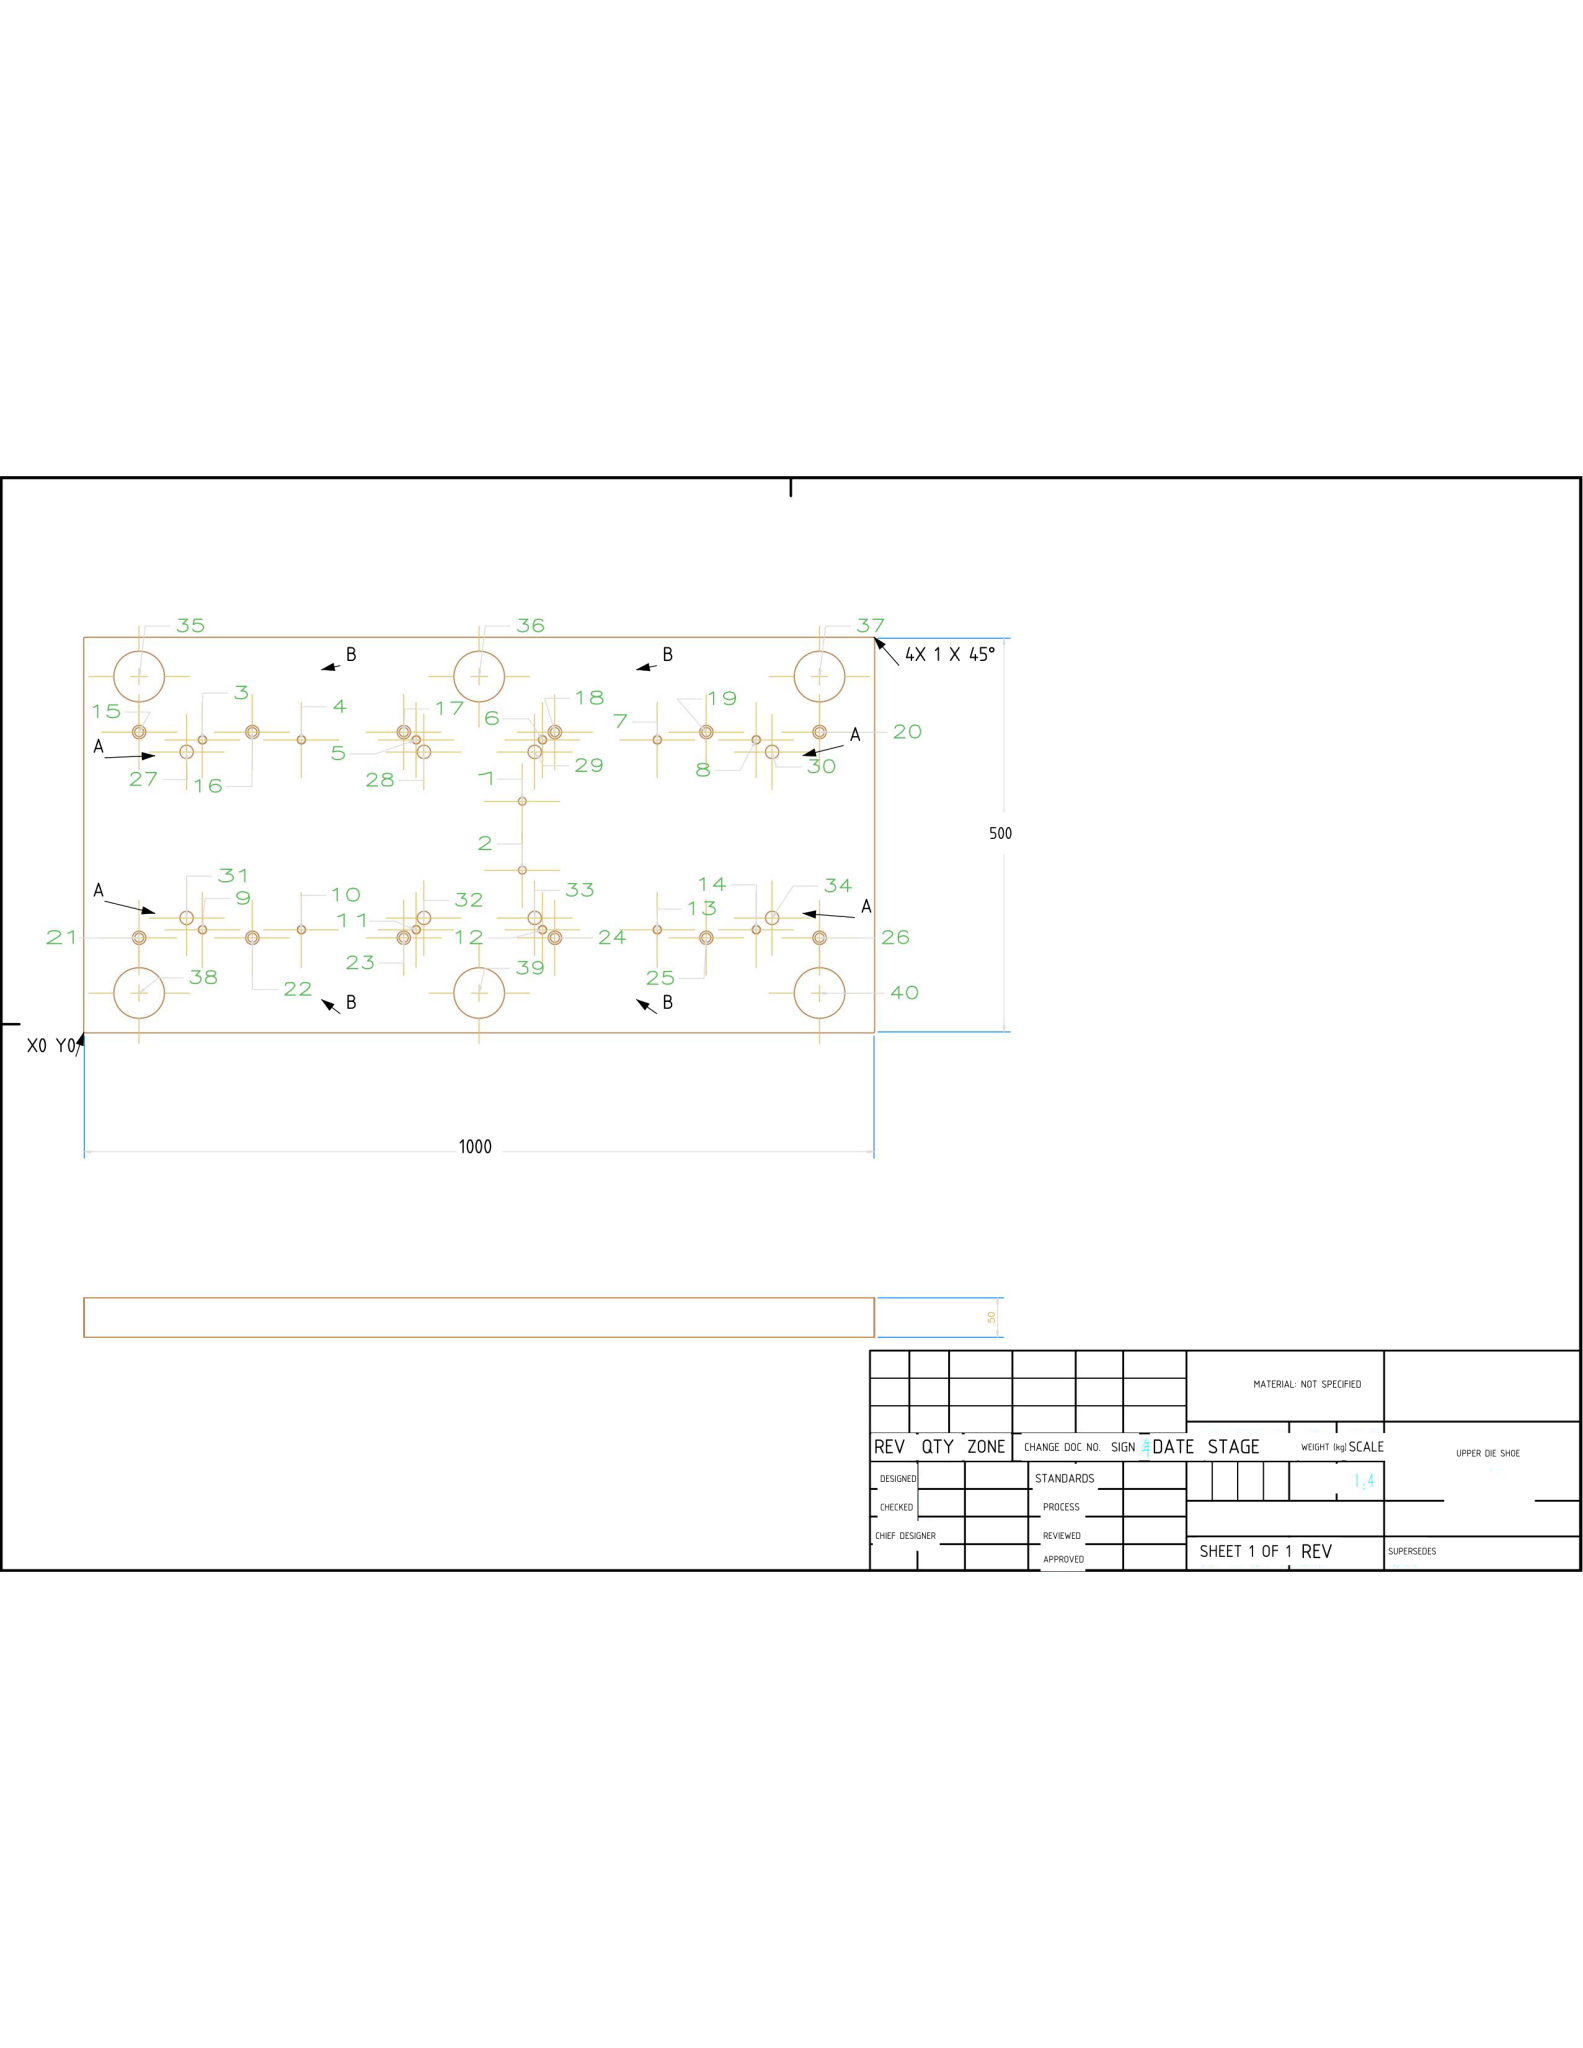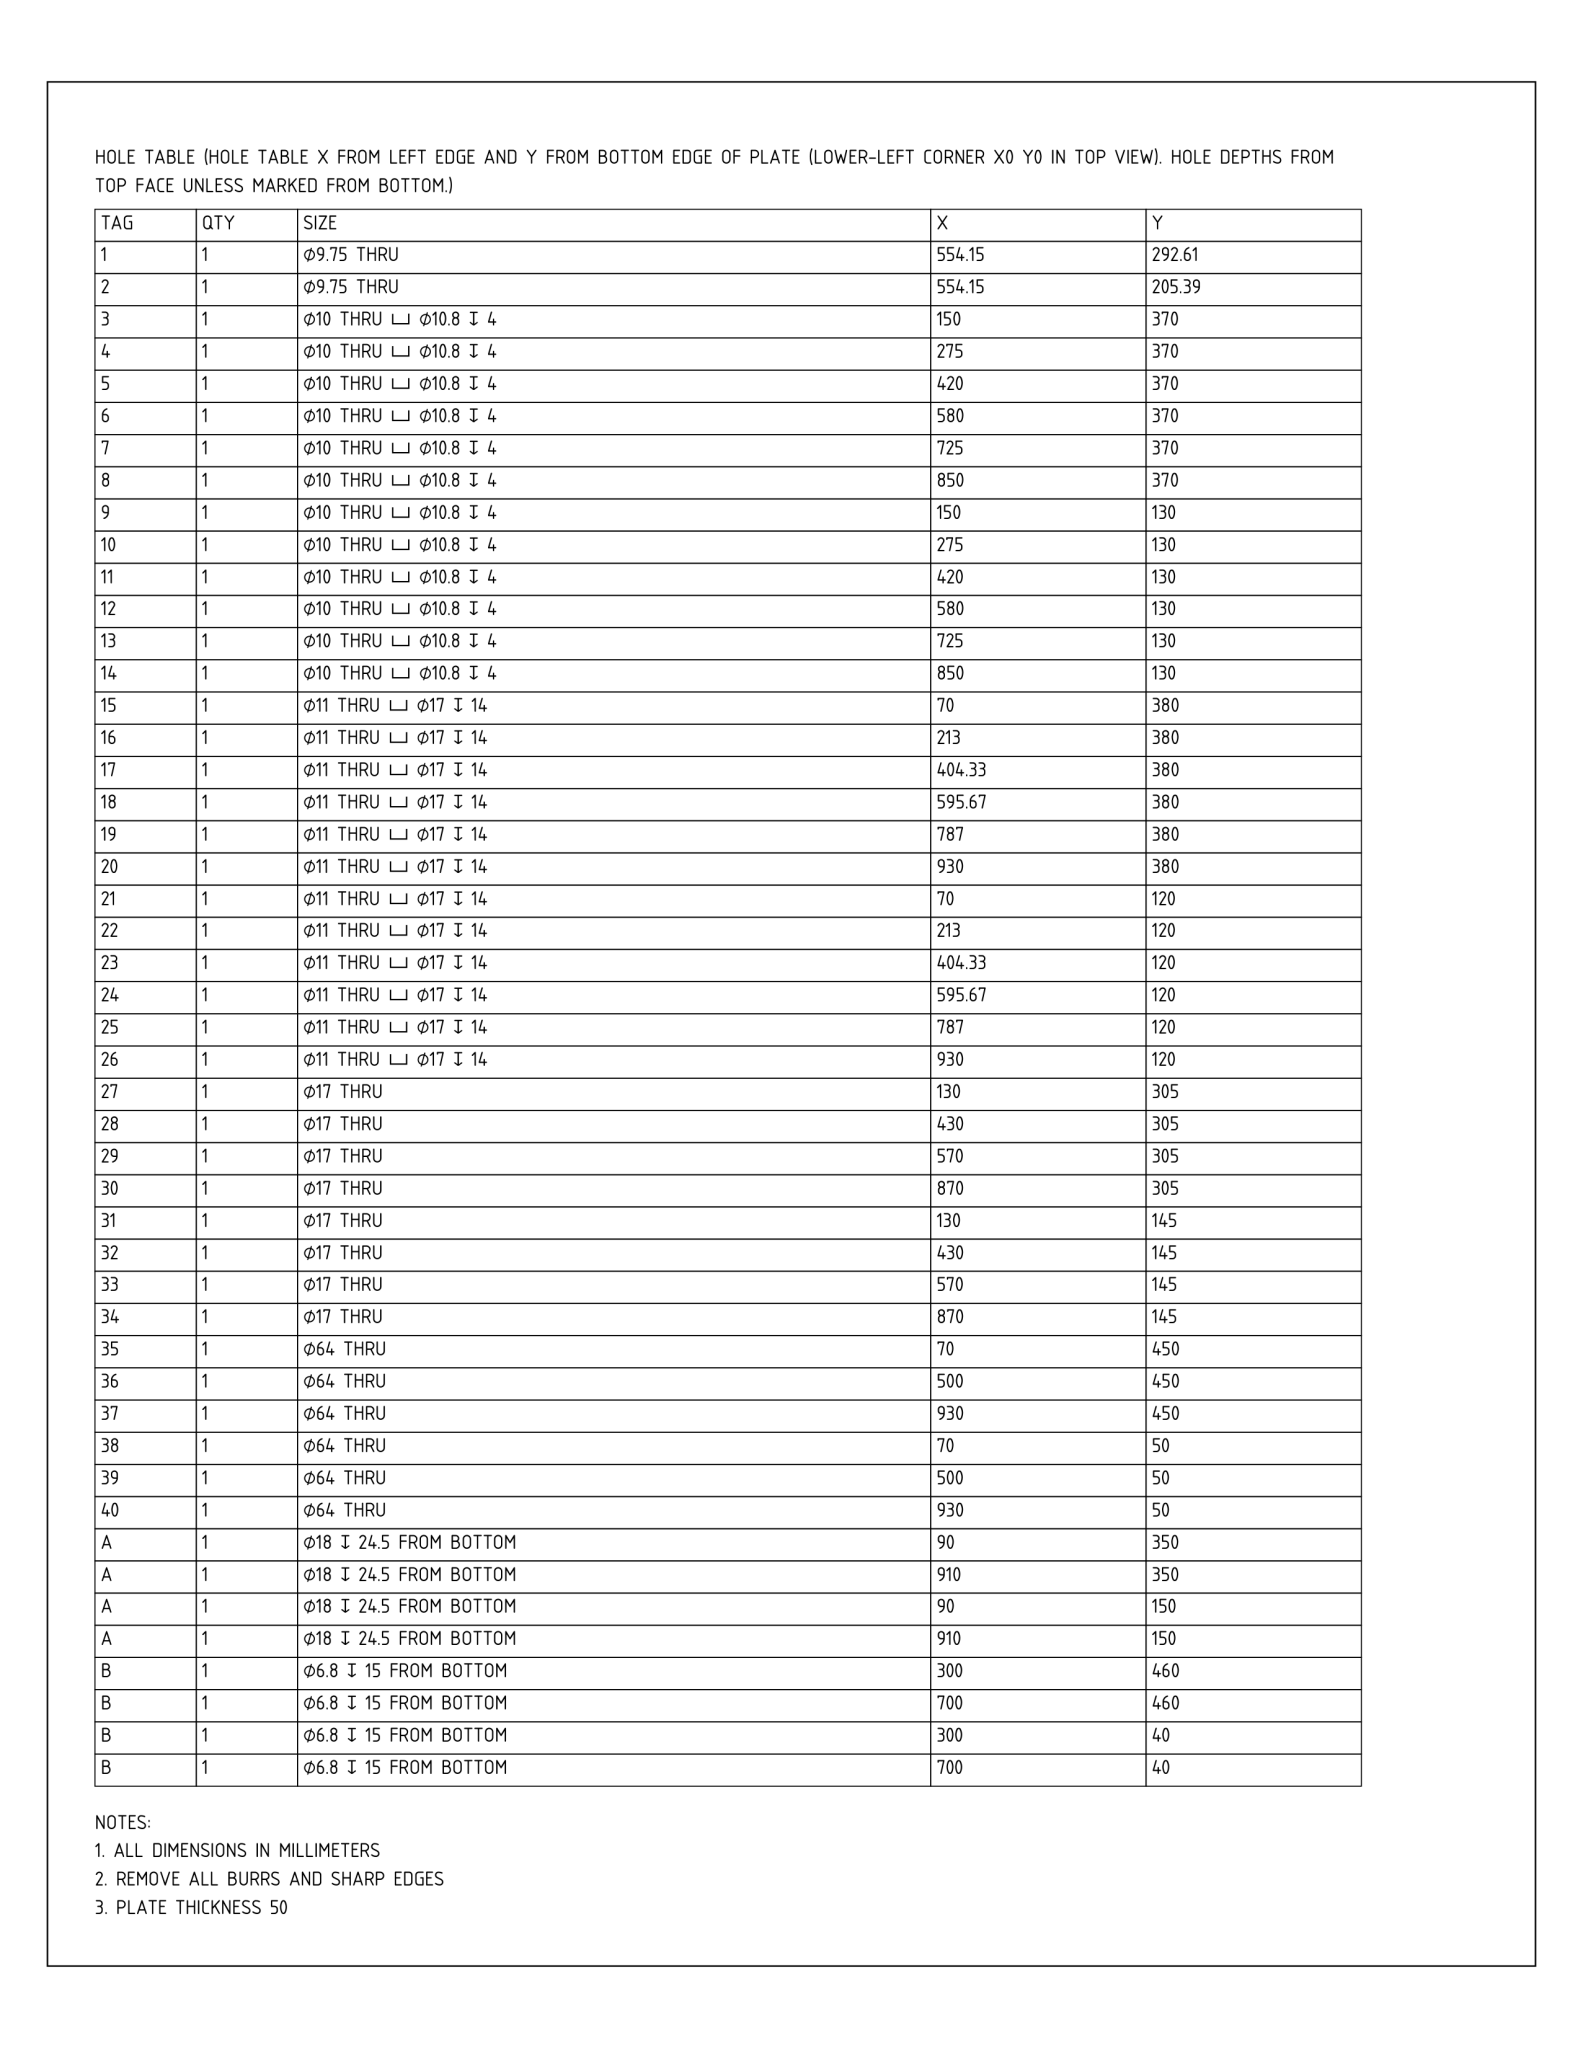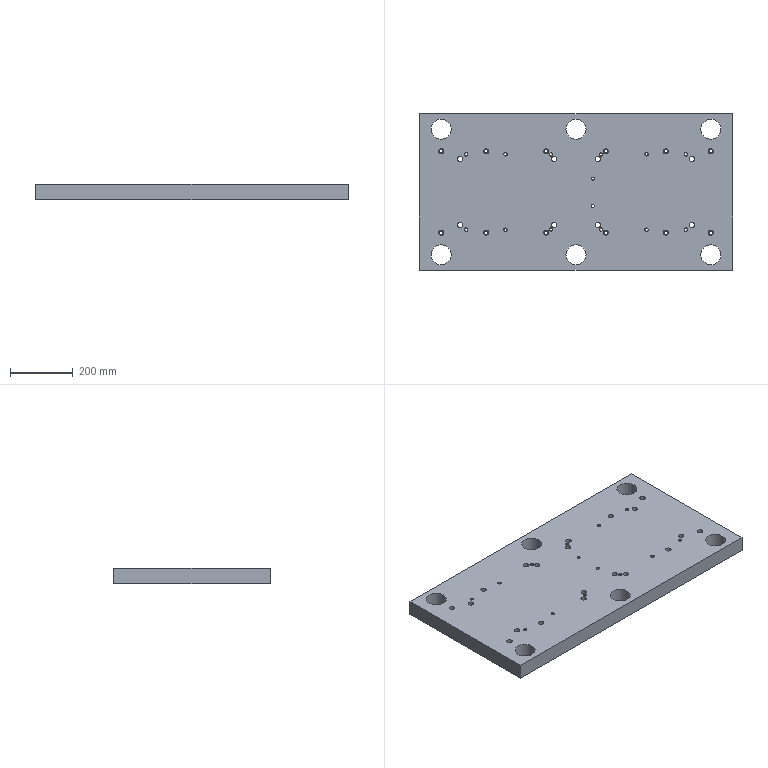Part | NX | mm | 1 solid | 114 faces | box 1000 x 500 x 50 mm | volume 23782489 mm3 | cylinder 72 | plane 42 | commonest cylinder face diameters 17 x20 11 x12 10.8 x12 10 x12 64 x6 6.8 x4 18 x4 9.75 x2